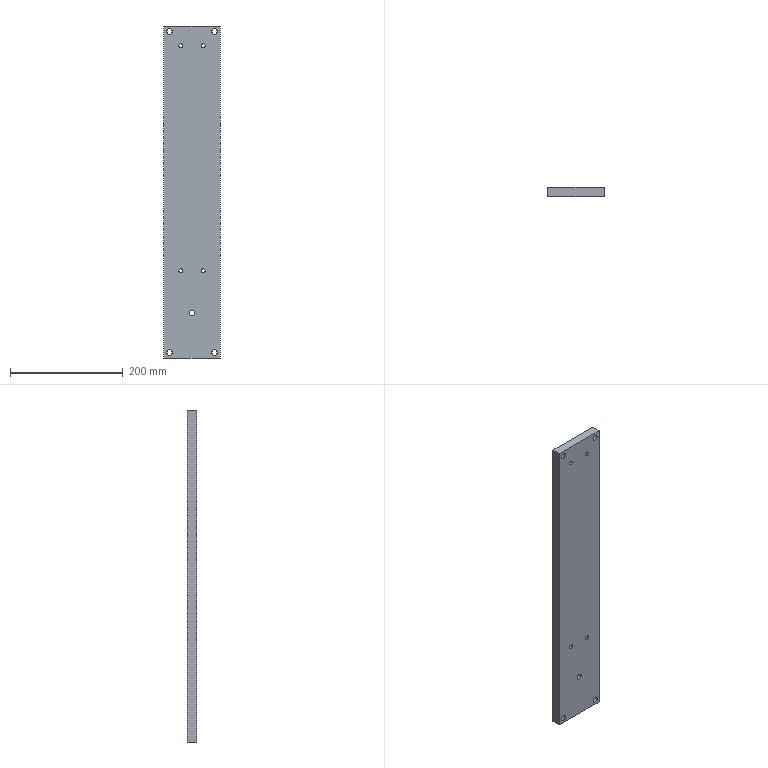Component | SolidWorks | TractionBasePlate-2 | 1 solid | 24 faces | box 100 x 16 x 590 mm | volume 935254 mm3 | cylinder 18 | plane 6 | commonest cylinder face diameters 10 x10 7 x8
build123d program:
from build123d import *

# Parameters (mm, degrees)
SKETCH1_W              = 590
SKETCH1_H              = 100
SKETCH1_R              = 5
SKETCH1_R_2            = 3.5
EXTRUDE1_DEPTH         = 16
M10_TAPPED_HOLE1_D     = 10
M10_TAPPED_HOLE1_DEPTH = 27.5
M10_TAPPED_HOLE1_TIP   = 3.004


with BuildPart() as part:
    # Sketch1 → Extrude1 (new body)
    with BuildSketch(Plane(origin=(0, 0, 0), x_dir=(1, 0, 0), z_dir=(0, 1, 0))):
        Rectangle(SKETCH1_W, SKETCH1_H)
        with Locations(Location((-285, 40, 0), (0, 0, 270))):
            Circle(SKETCH1_R, mode=Mode.SUBTRACT)
        with Locations(Location((-285, -40, 0), (0, 0, 270))):
            Circle(SKETCH1_R, mode=Mode.SUBTRACT)
        with Locations(Location((285, 40, 0), (0, 0, 270))):
            Circle(SKETCH1_R, mode=Mode.SUBTRACT)
        with Locations(Location((285, -40, 0), (0, 0, 270))):
            Circle(SKETCH1_R, mode=Mode.SUBTRACT)
        with Locations(Location((-260, 20, 0), (0, 0, 270))):
            Circle(SKETCH1_R_2, mode=Mode.SUBTRACT)
        with Locations(Location((-260, -20, 0), (0, 0, 270))):
            Circle(SKETCH1_R_2, mode=Mode.SUBTRACT)
        with Locations(Location((140, 20, 0), (0, 0, 270))):
            Circle(SKETCH1_R_2, mode=Mode.SUBTRACT)
        with Locations(Location((140, -20, 0), (0, 0, 270))):
            Circle(SKETCH1_R_2, mode=Mode.SUBTRACT)
    extrude(amount=EXTRUDE1_DEPTH)

    # M10 Tapped Hole1
    with Locations(Plane(origin=(0, 16, 0), x_dir=(-1, 0, 0), z_dir=(0, 1, 0))):
        with Locations((-215, 0)):
            Hole(M10_TAPPED_HOLE1_D / 2, depth=M10_TAPPED_HOLE1_DEPTH)
            with Locations((0, 0, -(M10_TAPPED_HOLE1_DEPTH + M10_TAPPED_HOLE1_TIP / 2))):  # 118° drill point
                Cone(0, M10_TAPPED_HOLE1_D / 2, M10_TAPPED_HOLE1_TIP, mode=Mode.SUBTRACT)


solid = part.part

# Placed as in the assembly
solid = solid.moved(Location((250.216, 370.983, 6.5), (0, 90, 0)))
STEP:
#1=CARTESIAN_POINT('',(9.654,14.606,-8.209));
#2=VERTEX_POINT('',#1);
#3=CARTESIAN_POINT('',(10.048,14.606,-8.209));
#4=VERTEX_POINT('',#3);
#5=CARTESIAN_POINT('',(9.851,14.606,-8.209));
#6=DIRECTION('',(0.,1.,0.));
#7=DIRECTION('',(1.,0.,0.));
#8=AXIS2_PLACEMENT_3D('',#5,#6,#7);
#9=CIRCLE('',#8,0.1969);
#10=EDGE_CURVE('',#2,#4,#9,.T.);
#11=ORIENTED_EDGE('',*,*,#10,.F.);
#12=CARTESIAN_POINT('',(9.654,15.236,-8.209));
#13=VERTEX_POINT('',#12);
#14=CARTESIAN_POINT('',(9.654,15.236,-8.209));
#15=DIRECTION('',(0.,1.,0.));
#16=VECTOR('',#15,39.37);
#17=LINE('',#14,#16);
#18=EDGE_CURVE('',#2,#13,#17,.T.);
#19=ORIENTED_EDGE('',*,*,#18,.T.);
#20=CARTESIAN_POINT('',(10.048,15.236,-8.209));
#21=VERTEX_POINT('',#20);
#22=CARTESIAN_POINT('',(9.851,15.236,-8.209));
#23=DIRECTION('',(0.,1.,0.));
#24=DIRECTION('',(1.,0.,0.));
#25=AXIS2_PLACEMENT_3D('',#22,#23,#24);
#26=CIRCLE('',#25,0.1969);
#27=EDGE_CURVE('',#13,#21,#26,.T.);
#28=ORIENTED_EDGE('',*,*,#27,.T.);
#29=CARTESIAN_POINT('',(10.048,15.236,-8.209));
#30=DIRECTION('',(0.,1.,0.));
#31=VECTOR('',#30,39.37);
#32=LINE('',#29,#31);
#33=EDGE_CURVE('',#4,#21,#32,.T.);
#34=ORIENTED_EDGE('',*,*,#33,.F.);
#35=EDGE_LOOP('',(#11,#19,#28,#34));
#36=FACE_OUTER_BOUND('',#35,.T.);
#37=CARTESIAN_POINT('',(9.851,15.236,-8.209));
#38=DIRECTION('',(0.,1.,0.));
#39=DIRECTION('',(1.,0.,0.));
#40=AXIS2_PLACEMENT_3D('',#37,#38,#39);
#41=CYLINDRICAL_SURFACE('',#40,0.1969);
#42=ADVANCED_FACE('',(#36),#41,.F.);
#43=CARTESIAN_POINT('',(10.501,15.236,-5.256));
#44=VERTEX_POINT('',#43);
#45=CARTESIAN_POINT('',(10.776,15.236,-5.256));
#46=VERTEX_POINT('',#45);
#47=CARTESIAN_POINT('',(10.638,15.236,-5.256));
#48=DIRECTION('',(0.,1.,0.));
#49=DIRECTION('',(1.,0.,0.));
#50=AXIS2_PLACEMENT_3D('',#47,#48,#49);
#51=CIRCLE('',#50,0.1378);
#52=EDGE_CURVE('',#44,#46,#51,.T.);
#53=ORIENTED_EDGE('',*,*,#52,.T.);
#54=CARTESIAN_POINT('',(10.776,14.606,-5.256));
#55=VERTEX_POINT('',#54);
#56=CARTESIAN_POINT('',(10.776,15.236,-5.256));
#57=DIRECTION('',(0.,-1.,0.));
#58=VECTOR('',#57,39.37);
#59=LINE('',#56,#58);
#60=EDGE_CURVE('',#46,#55,#59,.T.);
#61=ORIENTED_EDGE('',*,*,#60,.T.);
#62=CARTESIAN_POINT('',(10.501,14.606,-5.256));
#63=VERTEX_POINT('',#62);
#64=CARTESIAN_POINT('',(10.638,14.606,-5.256));
#65=DIRECTION('',(0.,1.,0.));
#66=DIRECTION('',(1.,0.,0.));
#67=AXIS2_PLACEMENT_3D('',#64,#65,#66);
#68=CIRCLE('',#67,0.1378);
#69=EDGE_CURVE('',#63,#55,#68,.T.);
#70=ORIENTED_EDGE('',*,*,#69,.F.);
#71=CARTESIAN_POINT('',(10.501,15.236,-5.256));
#72=DIRECTION('',(0.,-1.,0.));
#73=VECTOR('',#72,39.37);
#74=LINE('',#71,#73);
#75=EDGE_CURVE('',#44,#63,#74,.T.);
#76=ORIENTED_EDGE('',*,*,#75,.F.);
#77=EDGE_LOOP('',(#53,#61,#70,#76));
#78=FACE_OUTER_BOUND('',#77,.T.);
#79=CARTESIAN_POINT('',(10.638,15.236,-5.256));
#80=DIRECTION('',(0.,-1.,0.));
#81=DIRECTION('',(-1.,0.,0.));
#82=AXIS2_PLACEMENT_3D('',#79,#80,#81);
#83=CYLINDRICAL_SURFACE('',#82,0.1378);
#84=ADVANCED_FACE('',(#78),#83,.F.);
#85=CARTESIAN_POINT('',(8.926,15.236,-5.256));
#86=VERTEX_POINT('',#85);
#87=CARTESIAN_POINT('',(9.201,15.236,-5.256));
#88=VERTEX_POINT('',#87);
#89=CARTESIAN_POINT('',(9.064,15.236,-5.256));
#90=DIRECTION('',(0.,1.,0.));
#91=DIRECTION('',(1.,0.,0.));
#92=AXIS2_PLACEMENT_3D('',#89,#90,#91);
#93=CIRCLE('',#92,0.1378);
#94=EDGE_CURVE('',#86,#88,#93,.T.);
#95=ORIENTED_EDGE('',*,*,#94,.T.);
#96=CARTESIAN_POINT('',(9.201,14.606,-5.256));
#97=VERTEX_POINT('',#96);
#98=CARTESIAN_POINT('',(9.201,15.236,-5.256));
#99=DIRECTION('',(0.,-1.,0.));
#100=VECTOR('',#99,39.37);
#101=LINE('',#98,#100);
#102=EDGE_CURVE('',#88,#97,#101,.T.);
#103=ORIENTED_EDGE('',*,*,#102,.T.);
#104=CARTESIAN_POINT('',(8.926,14.606,-5.256));
#105=VERTEX_POINT('',#104);
#106=CARTESIAN_POINT('',(9.064,14.606,-5.256));
#107=DIRECTION('',(0.,1.,0.));
#108=DIRECTION('',(1.,0.,0.));
#109=AXIS2_PLACEMENT_3D('',#106,#107,#108);
#110=CIRCLE('',#109,0.1378);
#111=EDGE_CURVE('',#105,#97,#110,.T.);
#112=ORIENTED_EDGE('',*,*,#111,.F.);
#113=CARTESIAN_POINT('',(8.926,15.236,-5.256));
#114=DIRECTION('',(0.,-1.,0.));
#115=VECTOR('',#114,39.37);
#116=LINE('',#113,#115);
#117=EDGE_CURVE('',#86,#105,#116,.T.);
#118=ORIENTED_EDGE('',*,*,#117,.F.);
#119=EDGE_LOOP('',(#95,#103,#112,#118));
#120=FACE_OUTER_BOUND('',#119,.T.);
#121=CARTESIAN_POINT('',(9.064,15.236,-5.256));
#122=DIRECTION('',(0.,-1.,0.));
#123=DIRECTION('',(-1.,0.,0.));
#124=AXIS2_PLACEMENT_3D('',#121,#122,#123);
#125=CYLINDRICAL_SURFACE('',#124,0.1378);
#126=ADVANCED_FACE('',(#120),#125,.F.);
#127=CARTESIAN_POINT('',(10.501,15.236,10.492));
#128=VERTEX_POINT('',#127);
#129=CARTESIAN_POINT('',(10.776,15.236,10.492));
#130=VERTEX_POINT('',#129);
#131=CARTESIAN_POINT('',(10.638,15.236,10.492));
#132=DIRECTION('',(0.,1.,0.));
#133=DIRECTION('',(1.,0.,0.));
#134=AXIS2_PLACEMENT_3D('',#131,#132,#133);
#135=CIRCLE('',#134,0.1378);
#136=EDGE_CURVE('',#128,#130,#135,.T.);
#137=ORIENTED_EDGE('',*,*,#136,.T.);
#138=CARTESIAN_POINT('',(10.776,14.606,10.492));
#139=VERTEX_POINT('',#138);
#140=CARTESIAN_POINT('',(10.776,15.236,10.492));
#141=DIRECTION('',(0.,-1.,0.));
#142=VECTOR('',#141,39.37);
#143=LINE('',#140,#142);
#144=EDGE_CURVE('',#130,#139,#143,.T.);
#145=ORIENTED_EDGE('',*,*,#144,.T.);
#146=CARTESIAN_POINT('',(10.501,14.606,10.492));
#147=VERTEX_POINT('',#146);
#148=CARTESIAN_POINT('',(10.638,14.606,10.492));
#149=DIRECTION('',(0.,1.,0.));
#150=DIRECTION('',(1.,0.,0.));
#151=AXIS2_PLACEMENT_3D('',#148,#149,#150);
#152=CIRCLE('',#151,0.1378);
#153=EDGE_CURVE('',#147,#139,#152,.T.);
#154=ORIENTED_EDGE('',*,*,#153,.F.);
#155=CARTESIAN_POINT('',(10.501,15.236,10.492));
#156=DIRECTION('',(0.,-1.,0.));
#157=VECTOR('',#156,39.37);
#158=LINE('',#155,#157);
#159=EDGE_CURVE('',#128,#147,#158,.T.);
#160=ORIENTED_EDGE('',*,*,#159,.F.);
#161=EDGE_LOOP('',(#137,#145,#154,#160));
#162=FACE_OUTER_BOUND('',#161,.T.);
#163=CARTESIAN_POINT('',(10.638,15.236,10.492));
#164=DIRECTION('',(0.,-1.,0.));
#165=DIRECTION('',(-1.,0.,0.));
#166=AXIS2_PLACEMENT_3D('',#163,#164,#165);
#167=CYLINDRICAL_SURFACE('',#166,0.1378);
#168=ADVANCED_FACE('',(#162),#167,.F.);
#169=CARTESIAN_POINT('',(8.926,15.236,10.492));
#170=VERTEX_POINT('',#169);
#171=CARTESIAN_POINT('',(9.201,15.236,10.492));
#172=VERTEX_POINT('',#171);
#173=CARTESIAN_POINT('',(9.064,15.236,10.492));
#174=DIRECTION('',(0.,1.,0.));
#175=DIRECTION('',(1.,0.,0.));
#176=AXIS2_PLACEMENT_3D('',#173,#174,#175);
#177=CIRCLE('',#176,0.1378);
#178=EDGE_CURVE('',#170,#172,#177,.T.);
#179=ORIENTED_EDGE('',*,*,#178,.T.);
#180=CARTESIAN_POINT('',(9.201,14.606,10.492));
#181=VERTEX_POINT('',#180);
#182=CARTESIAN_POINT('',(9.201,15.236,10.492));
#183=DIRECTION('',(0.,-1.,0.));
#184=VECTOR('',#183,39.37);
#185=LINE('',#182,#184);
#186=EDGE_CURVE('',#172,#181,#185,.T.);
#187=ORIENTED_EDGE('',*,*,#186,.T.);
#188=CARTESIAN_POINT('',(8.926,14.606,10.492));
#189=VERTEX_POINT('',#188);
#190=CARTESIAN_POINT('',(9.064,14.606,10.492));
#191=DIRECTION('',(0.,1.,0.));
#192=DIRECTION('',(1.,0.,0.));
#193=AXIS2_PLACEMENT_3D('',#190,#191,#192);
#194=CIRCLE('',#193,0.1378);
#195=EDGE_CURVE('',#189,#181,#194,.T.);
#196=ORIENTED_EDGE('',*,*,#195,.F.);
#197=CARTESIAN_POINT('',(8.926,15.236,10.492));
#198=DIRECTION('',(0.,-1.,0.));
#199=VECTOR('',#198,39.37);
#200=LINE('',#197,#199);
#201=EDGE_CURVE('',#170,#189,#200,.T.);
#202=ORIENTED_EDGE('',*,*,#201,.F.);
#203=EDGE_LOOP('',(#179,#187,#196,#202));
#204=FACE_OUTER_BOUND('',#203,.T.);
#205=CARTESIAN_POINT('',(9.064,15.236,10.492));
#206=DIRECTION('',(0.,-1.,0.));
#207=DIRECTION('',(-1.,0.,0.));
#208=AXIS2_PLACEMENT_3D('',#205,#206,#207);
#209=CYLINDRICAL_SURFACE('',#208,0.1378);
#210=ADVANCED_FACE('',(#204),#209,.F.);
#211=CARTESIAN_POINT('',(11.229,15.236,-10.965));
#212=VERTEX_POINT('',#211);
#213=CARTESIAN_POINT('',(11.623,15.236,-10.965));
#214=VERTEX_POINT('',#213);
#215=CARTESIAN_POINT('',(11.426,15.236,-10.965));
#216=DIRECTION('',(0.,1.,0.));
#217=DIRECTION('',(1.,0.,0.));
#218=AXIS2_PLACEMENT_3D('',#215,#216,#217);
#219=CIRCLE('',#218,0.1969);
#220=EDGE_CURVE('',#212,#214,#219,.T.);
#221=ORIENTED_EDGE('',*,*,#220,.T.);
#222=CARTESIAN_POINT('',(11.623,14.606,-10.965));
#223=VERTEX_POINT('',#222);
#224=CARTESIAN_POINT('',(11.623,15.236,-10.965));
#225=DIRECTION('',(0.,-1.,0.));
#226=VECTOR('',#225,39.37);
#227=LINE('',#224,#226);
#228=EDGE_CURVE('',#214,#223,#227,.T.);
#229=ORIENTED_EDGE('',*,*,#228,.T.);
#230=CARTESIAN_POINT('',(11.229,14.606,-10.965));
#231=VERTEX_POINT('',#230);
#232=CARTESIAN_POINT('',(11.426,14.606,-10.965));
#233=DIRECTION('',(0.,1.,0.));
#234=DIRECTION('',(1.,0.,0.));
#235=AXIS2_PLACEMENT_3D('',#232,#233,#234);
#236=CIRCLE('',#235,0.1969);
#237=EDGE_CURVE('',#231,#223,#236,.T.);
#238=ORIENTED_EDGE('',*,*,#237,.F.);
#239=CARTESIAN_POINT('',(11.229,15.236,-10.965));
#240=DIRECTION('',(0.,-1.,0.));
#241=VECTOR('',#240,39.37);
#242=LINE('',#239,#241);
#243=EDGE_CURVE('',#212,#231,#242,.T.);
#244=ORIENTED_EDGE('',*,*,#243,.F.);
#245=EDGE_LOOP('',(#221,#229,#238,#244));
#246=FACE_OUTER_BOUND('',#245,.T.);
#247=CARTESIAN_POINT('',(11.426,15.236,-10.965));
#248=DIRECTION('',(0.,-1.,0.));
#249=DIRECTION('',(-1.,0.,0.));
#250=AXIS2_PLACEMENT_3D('',#247,#248,#249);
#251=CYLINDRICAL_SURFACE('',#250,0.1969);
#252=ADVANCED_FACE('',(#246),#251,.F.);
#253=CARTESIAN_POINT('',(8.079,15.236,-10.965));
#254=VERTEX_POINT('',#253);
#255=CARTESIAN_POINT('',(8.473,15.236,-10.965));
#256=VERTEX_POINT('',#255);
#257=CARTESIAN_POINT('',(8.276,15.236,-10.965));
#258=DIRECTION('',(0.,1.,0.));
#259=DIRECTION('',(1.,0.,0.));
#260=AXIS2_PLACEMENT_3D('',#257,#258,#259);
#261=CIRCLE('',#260,0.1969);
#262=EDGE_CURVE('',#254,#256,#261,.T.);
#263=ORIENTED_EDGE('',*,*,#262,.T.);
#264=CARTESIAN_POINT('',(8.473,14.606,-10.965));
#265=VERTEX_POINT('',#264);
#266=CARTESIAN_POINT('',(8.473,15.236,-10.965));
#267=DIRECTION('',(0.,-1.,0.));
#268=VECTOR('',#267,39.37);
#269=LINE('',#266,#268);
#270=EDGE_CURVE('',#256,#265,#269,.T.);
#271=ORIENTED_EDGE('',*,*,#270,.T.);
#272=CARTESIAN_POINT('',(8.079,14.606,-10.965));
#273=VERTEX_POINT('',#272);
#274=CARTESIAN_POINT('',(8.276,14.606,-10.965));
#275=DIRECTION('',(0.,1.,0.));
#276=DIRECTION('',(1.,0.,0.));
#277=AXIS2_PLACEMENT_3D('',#274,#275,#276);
#278=CIRCLE('',#277,0.1969);
#279=EDGE_CURVE('',#273,#265,#278,.T.);
#280=ORIENTED_EDGE('',*,*,#279,.F.);
#281=CARTESIAN_POINT('',(8.079,15.236,-10.965));
#282=DIRECTION('',(0.,-1.,0.));
#283=VECTOR('',#282,39.37);
#284=LINE('',#281,#283);
#285=EDGE_CURVE('',#254,#273,#284,.T.);
#286=ORIENTED_EDGE('',*,*,#285,.F.);
#287=EDGE_LOOP('',(#263,#271,#280,#286));
#288=FACE_OUTER_BOUND('',#287,.T.);
#289=CARTESIAN_POINT('',(8.276,15.236,-10.965));
#290=DIRECTION('',(0.,-1.,0.));
#291=DIRECTION('',(-1.,0.,0.));
#292=AXIS2_PLACEMENT_3D('',#289,#290,#291);
#293=CYLINDRICAL_SURFACE('',#292,0.1969);
#294=ADVANCED_FACE('',(#288),#293,.F.);
#295=CARTESIAN_POINT('',(11.229,15.236,11.476));
#296=VERTEX_POINT('',#295);
#297=CARTESIAN_POINT('',(11.623,15.236,11.476));
#298=VERTEX_POINT('',#297);
#299=CARTESIAN_POINT('',(11.426,15.236,11.476));
#300=DIRECTION('',(0.,1.,0.));
#301=DIRECTION('',(1.,0.,0.));
#302=AXIS2_PLACEMENT_3D('',#299,#300,#301);
#303=CIRCLE('',#302,0.1969);
#304=EDGE_CURVE('',#296,#298,#303,.T.);
#305=ORIENTED_EDGE('',*,*,#304,.T.);
#306=CARTESIAN_POINT('',(11.623,14.606,11.476));
#307=VERTEX_POINT('',#306);
#308=CARTESIAN_POINT('',(11.623,15.236,11.476));
#309=DIRECTION('',(0.,-1.,0.));
#310=VECTOR('',#309,39.37);
#311=LINE('',#308,#310);
#312=EDGE_CURVE('',#298,#307,#311,.T.);
#313=ORIENTED_EDGE('',*,*,#312,.T.);
#314=CARTESIAN_POINT('',(11.229,14.606,11.476));
#315=VERTEX_POINT('',#314);
#316=CARTESIAN_POINT('',(11.426,14.606,11.476));
#317=DIRECTION('',(0.,1.,0.));
#318=DIRECTION('',(1.,0.,0.));
#319=AXIS2_PLACEMENT_3D('',#316,#317,#318);
#320=CIRCLE('',#319,0.1969);
#321=EDGE_CURVE('',#315,#307,#320,.T.);
#322=ORIENTED_EDGE('',*,*,#321,.F.);
#323=CARTESIAN_POINT('',(11.229,15.236,11.476));
#324=DIRECTION('',(0.,-1.,0.));
#325=VECTOR('',#324,39.37);
#326=LINE('',#323,#325);
#327=EDGE_CURVE('',#296,#315,#326,.T.);
#328=ORIENTED_EDGE('',*,*,#327,.F.);
#329=EDGE_LOOP('',(#305,#313,#322,#328));
#330=FACE_OUTER_BOUND('',#329,.T.);
#331=CARTESIAN_POINT('',(11.426,15.236,11.476));
#332=DIRECTION('',(0.,-1.,0.));
#333=DIRECTION('',(-1.,0.,0.));
#334=AXIS2_PLACEMENT_3D('',#331,#332,#333);
#335=CYLINDRICAL_SURFACE('',#334,0.1969);
#336=ADVANCED_FACE('',(#330),#335,.F.);
#337=CARTESIAN_POINT('',(8.079,15.236,11.476));
#338=VERTEX_POINT('',#337);
#339=CARTESIAN_POINT('',(8.473,15.236,11.476));
#340=VERTEX_POINT('',#339);
#341=CARTESIAN_POINT('',(8.276,15.236,11.476));
#342=DIRECTION('',(0.,1.,0.));
#343=DIRECTION('',(1.,0.,0.));
#344=AXIS2_PLACEMENT_3D('',#341,#342,#343);
#345=CIRCLE('',#344,0.1969);
#346=EDGE_CURVE('',#338,#340,#345,.T.);
#347=ORIENTED_EDGE('',*,*,#346,.T.);
#348=CARTESIAN_POINT('',(8.473,14.606,11.476));
#349=VERTEX_POINT('',#348);
#350=CARTESIAN_POINT('',(8.473,15.236,11.476));
#351=DIRECTION('',(0.,-1.,0.));
#352=VECTOR('',#351,39.37);
#353=LINE('',#350,#352);
#354=EDGE_CURVE('',#340,#349,#353,.T.);
#355=ORIENTED_EDGE('',*,*,#354,.T.);
#356=CARTESIAN_POINT('',(8.079,14.606,11.476));
#357=VERTEX_POINT('',#356);
#358=CARTESIAN_POINT('',(8.276,14.606,11.476));
#359=DIRECTION('',(0.,1.,0.));
#360=DIRECTION('',(1.,0.,0.));
#361=AXIS2_PLACEMENT_3D('',#358,#359,#360);
#362=CIRCLE('',#361,0.1969);
#363=EDGE_CURVE('',#357,#349,#362,.T.);
#364=ORIENTED_EDGE('',*,*,#363,.F.);
#365=CARTESIAN_POINT('',(8.079,15.236,11.476));
#366=DIRECTION('',(0.,-1.,0.));
#367=VECTOR('',#366,39.37);
#368=LINE('',#365,#367);
#369=EDGE_CURVE('',#338,#357,#368,.T.);
#370=ORIENTED_EDGE('',*,*,#369,.F.);
#371=EDGE_LOOP('',(#347,#355,#364,#370));
#372=FACE_OUTER_BOUND('',#371,.T.);
#373=CARTESIAN_POINT('',(8.276,15.236,11.476));
#374=DIRECTION('',(0.,-1.,0.));
#375=DIRECTION('',(-1.,0.,0.));
#376=AXIS2_PLACEMENT_3D('',#373,#374,#375);
#377=CYLINDRICAL_SURFACE('',#376,0.1969);
#378=ADVANCED_FACE('',(#372),#377,.F.);
#379=CARTESIAN_POINT('',(9.851,15.236,-8.209));
#380=DIRECTION('',(0.,1.,0.));
#381=DIRECTION('',(1.,0.,0.));
#382=AXIS2_PLACEMENT_3D('',#379,#380,#381);
#383=CIRCLE('',#382,0.1969);
#384=EDGE_CURVE('',#21,#13,#383,.T.);
#385=ORIENTED_EDGE('',*,*,#384,.F.);
#386=ORIENTED_EDGE('',*,*,#27,.F.);
#387=EDGE_LOOP('',(#385,#386));
#388=FACE_BOUND('',#387,.T.);
#389=ORIENTED_EDGE('',*,*,#94,.F.);
#390=CARTESIAN_POINT('',(9.064,15.236,-5.256));
#391=DIRECTION('',(0.,1.,0.));
#392=DIRECTION('',(1.,0.,0.));
#393=AXIS2_PLACEMENT_3D('',#390,#391,#392);
#394=CIRCLE('',#393,0.1378);
#395=EDGE_CURVE('',#88,#86,#394,.T.);
#396=ORIENTED_EDGE('',*,*,#395,.F.);
#397=EDGE_LOOP('',(#389,#396));
#398=FACE_BOUND('',#397,.T.);
#399=ORIENTED_EDGE('',*,*,#178,.F.);
#400=CARTESIAN_POINT('',(9.064,15.236,10.492));
#401=DIRECTION('',(0.,1.,0.));
#402=DIRECTION('',(1.,0.,0.));
#403=AXIS2_PLACEMENT_3D('',#400,#401,#402);
#404=CIRCLE('',#403,0.1378);
#405=EDGE_CURVE('',#172,#170,#404,.T.);
#406=ORIENTED_EDGE('',*,*,#405,.F.);
#407=EDGE_LOOP('',(#399,#406));
#408=FACE_BOUND('',#407,.T.);
#409=ORIENTED_EDGE('',*,*,#262,.F.);
#410=CARTESIAN_POINT('',(8.276,15.236,-10.965));
#411=DIRECTION('',(0.,1.,0.));
#412=DIRECTION('',(1.,0.,0.));
#413=AXIS2_PLACEMENT_3D('',#410,#411,#412);
#414=CIRCLE('',#413,0.1969);
#415=EDGE_CURVE('',#256,#254,#414,.T.);
#416=ORIENTED_EDGE('',*,*,#415,.F.);
#417=EDGE_LOOP('',(#409,#416));
#418=FACE_BOUND('',#417,.T.);
#419=ORIENTED_EDGE('',*,*,#346,.F.);
#420=CARTESIAN_POINT('',(8.276,15.236,11.476));
#421=DIRECTION('',(0.,1.,0.));
#422=DIRECTION('',(1.,0.,0.));
#423=AXIS2_PLACEMENT_3D('',#420,#421,#422);
#424=CIRCLE('',#423,0.1969);
#425=EDGE_CURVE('',#340,#338,#424,.T.);
#426=ORIENTED_EDGE('',*,*,#425,.F.);
#427=EDGE_LOOP('',(#419,#426));
#428=FACE_BOUND('',#427,.T.);
#429=CARTESIAN_POINT('',(7.883,15.236,11.87));
#430=VERTEX_POINT('',#429);
#431=CARTESIAN_POINT('',(11.82,15.236,11.87));
#432=VERTEX_POINT('',#431);
#433=CARTESIAN_POINT('',(7.883,15.236,11.87));
#434=DIRECTION('',(1.,0.,0.));
#435=VECTOR('',#434,39.37);
#436=LINE('',#433,#435);
#437=EDGE_CURVE('',#430,#432,#436,.T.);
#438=ORIENTED_EDGE('',*,*,#437,.T.);
#439=CARTESIAN_POINT('',(11.82,15.236,-11.358));
#440=VERTEX_POINT('',#439);
#441=CARTESIAN_POINT('',(11.82,15.236,11.87));
#442=DIRECTION('',(0.,0.,-1.));
#443=VECTOR('',#442,39.37);
#444=LINE('',#441,#443);
#445=EDGE_CURVE('',#432,#440,#444,.T.);
#446=ORIENTED_EDGE('',*,*,#445,.T.);
#447=CARTESIAN_POINT('',(7.883,15.236,-11.358));
#448=VERTEX_POINT('',#447);
#449=CARTESIAN_POINT('',(7.883,15.236,-11.358));
#450=DIRECTION('',(-1.,0.,0.));
#451=VECTOR('',#450,39.37);
#452=LINE('',#449,#451);
#453=EDGE_CURVE('',#440,#448,#452,.T.);
#454=ORIENTED_EDGE('',*,*,#453,.T.);
#455=CARTESIAN_POINT('',(7.883,15.236,11.87));
#456=DIRECTION('',(0.,0.,1.));
#457=VECTOR('',#456,39.37);
#458=LINE('',#455,#457);
#459=EDGE_CURVE('',#448,#430,#458,.T.);
#460=ORIENTED_EDGE('',*,*,#459,.T.);
#461=EDGE_LOOP('',(#438,#446,#454,#460));
#462=FACE_OUTER_BOUND('',#461,.T.);
#463=ORIENTED_EDGE('',*,*,#304,.F.);
#464=CARTESIAN_POINT('',(11.426,15.236,11.476));
#465=DIRECTION('',(0.,1.,0.));
#466=DIRECTION('',(1.,0.,0.));
#467=AXIS2_PLACEMENT_3D('',#464,#465,#466);
#468=CIRCLE('',#467,0.1969);
#469=EDGE_CURVE('',#298,#296,#468,.T.);
#470=ORIENTED_EDGE('',*,*,#469,.F.);
#471=EDGE_LOOP('',(#463,#470));
#472=FACE_BOUND('',#471,.T.);
#473=ORIENTED_EDGE('',*,*,#220,.F.);
#474=CARTESIAN_POINT('',(11.426,15.236,-10.965));
#475=DIRECTION('',(0.,1.,0.));
#476=DIRECTION('',(1.,0.,0.));
#477=AXIS2_PLACEMENT_3D('',#474,#475,#476);
#478=CIRCLE('',#477,0.1969);
#479=EDGE_CURVE('',#214,#212,#478,.T.);
#480=ORIENTED_EDGE('',*,*,#479,.F.);
#481=EDGE_LOOP('',(#473,#480));
#482=FACE_BOUND('',#481,.T.);
#483=ORIENTED_EDGE('',*,*,#136,.F.);
#484=CARTESIAN_POINT('',(10.638,15.236,10.492));
#485=DIRECTION('',(0.,1.,0.));
#486=DIRECTION('',(1.,0.,0.));
#487=AXIS2_PLACEMENT_3D('',#484,#485,#486);
#488=CIRCLE('',#487,0.1378);
#489=EDGE_CURVE('',#130,#128,#488,.T.);
#490=ORIENTED_EDGE('',*,*,#489,.F.);
#491=EDGE_LOOP('',(#483,#490));
#492=FACE_BOUND('',#491,.T.);
#493=ORIENTED_EDGE('',*,*,#52,.F.);
#494=CARTESIAN_POINT('',(10.638,15.236,-5.256));
#495=DIRECTION('',(0.,1.,0.));
#496=DIRECTION('',(1.,0.,0.));
#497=AXIS2_PLACEMENT_3D('',#494,#495,#496);
#498=CIRCLE('',#497,0.1378);
#499=EDGE_CURVE('',#46,#44,#498,.T.);
#500=ORIENTED_EDGE('',*,*,#499,.F.);
#501=EDGE_LOOP('',(#493,#500));
#502=FACE_BOUND('',#501,.T.);
#503=CARTESIAN_POINT('',(11.82,15.236,11.87));
#504=DIRECTION('',(0.,1.,0.));
#505=DIRECTION('',(1.,0.,0.));
#506=AXIS2_PLACEMENT_3D('',#503,#504,#505);
#507=PLANE('',#506);
#508=ADVANCED_FACE('',(#388,#398,#408,#418,#428,#462,#472,#482,#492,#502),#507,.T.);
#509=CARTESIAN_POINT('',(9.851,14.606,-8.209));
#510=DIRECTION('',(0.,1.,0.));
#511=DIRECTION('',(1.,0.,0.));
#512=AXIS2_PLACEMENT_3D('',#509,#510,#511);
#513=CIRCLE('',#512,0.1969);
#514=EDGE_CURVE('',#4,#2,#513,.T.);
#515=ORIENTED_EDGE('',*,*,#514,.T.);
#516=ORIENTED_EDGE('',*,*,#10,.T.);
#517=EDGE_LOOP('',(#515,#516));
#518=FACE_BOUND('',#517,.T.);
#519=CARTESIAN_POINT('',(7.883,14.606,11.87));
#520=VERTEX_POINT('',#519);
#521=CARTESIAN_POINT('',(11.82,14.606,11.87));
#522=VERTEX_POINT('',#521);
#523=CARTESIAN_POINT('',(7.883,14.606,11.87));
#524=DIRECTION('',(1.,0.,0.));
#525=VECTOR('',#524,39.37);
#526=LINE('',#523,#525);
#527=EDGE_CURVE('',#520,#522,#526,.T.);
#528=ORIENTED_EDGE('',*,*,#527,.F.);
#529=CARTESIAN_POINT('',(7.883,14.606,-11.358));
#530=VERTEX_POINT('',#529);
#531=CARTESIAN_POINT('',(7.883,14.606,11.87));
#532=DIRECTION('',(0.,0.,1.));
#533=VECTOR('',#532,39.37);
#534=LINE('',#531,#533);
#535=EDGE_CURVE('',#530,#520,#534,.T.);
#536=ORIENTED_EDGE('',*,*,#535,.F.);
#537=CARTESIAN_POINT('',(11.82,14.606,-11.358));
#538=VERTEX_POINT('',#537);
#539=CARTESIAN_POINT('',(7.883,14.606,-11.358));
#540=DIRECTION('',(-1.,0.,0.));
#541=VECTOR('',#540,39.37);
#542=LINE('',#539,#541);
#543=EDGE_CURVE('',#538,#530,#542,.T.);
#544=ORIENTED_EDGE('',*,*,#543,.F.);
#545=CARTESIAN_POINT('',(11.82,14.606,11.87));
#546=DIRECTION('',(0.,0.,-1.));
#547=VECTOR('',#546,39.37);
#548=LINE('',#545,#547);
#549=EDGE_CURVE('',#522,#538,#548,.T.);
#550=ORIENTED_EDGE('',*,*,#549,.F.);
#551=EDGE_LOOP('',(#528,#536,#544,#550));
#552=FACE_OUTER_BOUND('',#551,.T.);
#553=ORIENTED_EDGE('',*,*,#363,.T.);
#554=CARTESIAN_POINT('',(8.276,14.606,11.476));
#555=DIRECTION('',(0.,1.,0.));
#556=DIRECTION('',(1.,0.,0.));
#557=AXIS2_PLACEMENT_3D('',#554,#555,#556);
#558=CIRCLE('',#557,0.1969);
#559=EDGE_CURVE('',#349,#357,#558,.T.);
#560=ORIENTED_EDGE('',*,*,#559,.T.);
#561=EDGE_LOOP('',(#553,#560));
#562=FACE_BOUND('',#561,.T.);
#563=ORIENTED_EDGE('',*,*,#321,.T.);
#564=CARTESIAN_POINT('',(11.426,14.606,11.476));
#565=DIRECTION('',(0.,1.,0.));
#566=DIRECTION('',(1.,0.,0.));
#567=AXIS2_PLACEMENT_3D('',#564,#565,#566);
#568=CIRCLE('',#567,0.1969);
#569=EDGE_CURVE('',#307,#315,#568,.T.);
#570=ORIENTED_EDGE('',*,*,#569,.T.);
#571=EDGE_LOOP('',(#563,#570));
#572=FACE_BOUND('',#571,.T.);
#573=ORIENTED_EDGE('',*,*,#279,.T.);
#574=CARTESIAN_POINT('',(8.276,14.606,-10.965));
#575=DIRECTION('',(0.,1.,0.));
#576=DIRECTION('',(1.,0.,0.));
#577=AXIS2_PLACEMENT_3D('',#574,#575,#576);
#578=CIRCLE('',#577,0.1969);
#579=EDGE_CURVE('',#265,#273,#578,.T.);
#580=ORIENTED_EDGE('',*,*,#579,.T.);
#581=EDGE_LOOP('',(#573,#580));
#582=FACE_BOUND('',#581,.T.);
#583=ORIENTED_EDGE('',*,*,#237,.T.);
#584=CARTESIAN_POINT('',(11.426,14.606,-10.965));
#585=DIRECTION('',(0.,1.,0.));
#586=DIRECTION('',(1.,0.,0.));
#587=AXIS2_PLACEMENT_3D('',#584,#585,#586);
#588=CIRCLE('',#587,0.1969);
#589=EDGE_CURVE('',#223,#231,#588,.T.);
#590=ORIENTED_EDGE('',*,*,#589,.T.);
#591=EDGE_LOOP('',(#583,#590));
#592=FACE_BOUND('',#591,.T.);
#593=ORIENTED_EDGE('',*,*,#195,.T.);
#594=CARTESIAN_POINT('',(9.064,14.606,10.492));
#595=DIRECTION('',(0.,1.,0.));
#596=DIRECTION('',(1.,0.,0.));
#597=AXIS2_PLACEMENT_3D('',#594,#595,#596);
#598=CIRCLE('',#597,0.1378);
#599=EDGE_CURVE('',#181,#189,#598,.T.);
#600=ORIENTED_EDGE('',*,*,#599,.T.);
#601=EDGE_LOOP('',(#593,#600));
#602=FACE_BOUND('',#601,.T.);
#603=ORIENTED_EDGE('',*,*,#153,.T.);
#604=CARTESIAN_POINT('',(10.638,14.606,10.492));
#605=DIRECTION('',(0.,1.,0.));
#606=DIRECTION('',(1.,0.,0.));
#607=AXIS2_PLACEMENT_3D('',#604,#605,#606);
#608=CIRCLE('',#607,0.1378);
#609=EDGE_CURVE('',#139,#147,#608,.T.);
#610=ORIENTED_EDGE('',*,*,#609,.T.);
#611=EDGE_LOOP('',(#603,#610));
#612=FACE_BOUND('',#611,.T.);
#613=ORIENTED_EDGE('',*,*,#111,.T.);
#614=CARTESIAN_POINT('',(9.064,14.606,-5.256));
#615=DIRECTION('',(0.,1.,0.));
#616=DIRECTION('',(1.,0.,0.));
#617=AXIS2_PLACEMENT_3D('',#614,#615,#616);
#618=CIRCLE('',#617,0.1378);
#619=EDGE_CURVE('',#97,#105,#618,.T.);
#620=ORIENTED_EDGE('',*,*,#619,.T.);
#621=EDGE_LOOP('',(#613,#620));
#622=FACE_BOUND('',#621,.T.);
#623=ORIENTED_EDGE('',*,*,#69,.T.);
#624=CARTESIAN_POINT('',(10.638,14.606,-5.256));
#625=DIRECTION('',(0.,1.,0.));
#626=DIRECTION('',(1.,0.,0.));
#627=AXIS2_PLACEMENT_3D('',#624,#625,#626);
#628=CIRCLE('',#627,0.1378);
#629=EDGE_CURVE('',#55,#63,#628,.T.);
#630=ORIENTED_EDGE('',*,*,#629,.T.);
#631=EDGE_LOOP('',(#623,#630));
#632=FACE_BOUND('',#631,.T.);
#633=CARTESIAN_POINT('',(11.82,14.606,11.87));
#634=DIRECTION('',(0.,1.,0.));
#635=DIRECTION('',(1.,0.,0.));
#636=AXIS2_PLACEMENT_3D('',#633,#634,#635);
#637=PLANE('',#636);
#638=ADVANCED_FACE('',(#518,#552,#562,#572,#582,#592,#602,#612,#622,#632),#637,.F.);
#639=ORIENTED_EDGE('',*,*,#527,.T.);
#640=CARTESIAN_POINT('',(11.82,15.236,11.87));
#641=DIRECTION('',(0.,-1.,0.));
#642=VECTOR('',#641,39.37);
#643=LINE('',#640,#642);
#644=EDGE_CURVE('',#432,#522,#643,.T.);
#645=ORIENTED_EDGE('',*,*,#644,.F.);
#646=ORIENTED_EDGE('',*,*,#437,.F.);
#647=CARTESIAN_POINT('',(7.883,15.236,11.87));
#648=DIRECTION('',(0.,-1.,0.));
#649=VECTOR('',#648,39.37);
#650=LINE('',#647,#649);
#651=EDGE_CURVE('',#430,#520,#650,.T.);
#652=ORIENTED_EDGE('',*,*,#651,.T.);
#653=EDGE_LOOP('',(#639,#645,#646,#652));
#654=FACE_OUTER_BOUND('',#653,.T.);
#655=CARTESIAN_POINT('',(7.883,15.236,11.87));
#656=DIRECTION('',(0.,0.,-1.));
#657=DIRECTION('',(-1.,0.,0.));
#658=AXIS2_PLACEMENT_3D('',#655,#656,#657);
#659=PLANE('',#658);
#660=ADVANCED_FACE('',(#654),#659,.F.);
#661=ORIENTED_EDGE('',*,*,#549,.T.);
#662=CARTESIAN_POINT('',(11.82,15.236,-11.358));
#663=DIRECTION('',(0.,-1.,0.));
#664=VECTOR('',#663,39.37);
#665=LINE('',#662,#664);
#666=EDGE_CURVE('',#440,#538,#665,.T.);
#667=ORIENTED_EDGE('',*,*,#666,.F.);
#668=ORIENTED_EDGE('',*,*,#445,.F.);
#669=ORIENTED_EDGE('',*,*,#644,.T.);
#670=EDGE_LOOP('',(#661,#667,#668,#669));
#671=FACE_OUTER_BOUND('',#670,.T.);
#672=CARTESIAN_POINT('',(11.82,15.236,11.87));
#673=DIRECTION('',(-1.,0.,0.));
#674=DIRECTION('',(0.,0.,1.));
#675=AXIS2_PLACEMENT_3D('',#672,#673,#674);
#676=PLANE('',#675);
#677=ADVANCED_FACE('',(#671),#676,.F.);
#678=ORIENTED_EDGE('',*,*,#543,.T.);
#679=CARTESIAN_POINT('',(7.883,15.236,-11.358));
#680=DIRECTION('',(0.,-1.,0.));
#681=VECTOR('',#680,39.37);
#682=LINE('',#679,#681);
#683=EDGE_CURVE('',#448,#530,#682,.T.);
#684=ORIENTED_EDGE('',*,*,#683,.F.);
#685=ORIENTED_EDGE('',*,*,#453,.F.);
#686=ORIENTED_EDGE('',*,*,#666,.T.);
#687=EDGE_LOOP('',(#678,#684,#685,#686));
#688=FACE_OUTER_BOUND('',#687,.T.);
#689=CARTESIAN_POINT('',(7.883,15.236,-11.358));
#690=DIRECTION('',(0.,0.,1.));
#691=DIRECTION('',(1.,0.,0.));
#692=AXIS2_PLACEMENT_3D('',#689,#690,#691);
#693=PLANE('',#692);
#694=ADVANCED_FACE('',(#688),#693,.F.);
#695=ORIENTED_EDGE('',*,*,#535,.T.);
#696=ORIENTED_EDGE('',*,*,#651,.F.);
#697=ORIENTED_EDGE('',*,*,#459,.F.);
#698=ORIENTED_EDGE('',*,*,#683,.T.);
#699=EDGE_LOOP('',(#695,#696,#697,#698));
#700=FACE_OUTER_BOUND('',#699,.T.);
#701=CARTESIAN_POINT('',(7.883,15.236,11.87));
#702=DIRECTION('',(1.,0.,0.));
#703=DIRECTION('',(0.,0.,-1.));
#704=AXIS2_PLACEMENT_3D('',#701,#702,#703);
#705=PLANE('',#704);
#706=ADVANCED_FACE('',(#700),#705,.F.);
#707=ORIENTED_EDGE('',*,*,#354,.F.);
#708=ORIENTED_EDGE('',*,*,#425,.T.);
#709=ORIENTED_EDGE('',*,*,#369,.T.);
#710=ORIENTED_EDGE('',*,*,#559,.F.);
#711=EDGE_LOOP('',(#707,#708,#709,#710));
#712=FACE_OUTER_BOUND('',#711,.T.);
#713=CARTESIAN_POINT('',(8.276,15.236,11.476));
#714=DIRECTION('',(0.,-1.,0.));
#715=DIRECTION('',(-1.,0.,0.));
#716=AXIS2_PLACEMENT_3D('',#713,#714,#715);
#717=CYLINDRICAL_SURFACE('',#716,0.1969);
#718=ADVANCED_FACE('',(#712),#717,.F.);
#719=ORIENTED_EDGE('',*,*,#312,.F.);
#720=ORIENTED_EDGE('',*,*,#469,.T.);
#721=ORIENTED_EDGE('',*,*,#327,.T.);
#722=ORIENTED_EDGE('',*,*,#569,.F.);
#723=EDGE_LOOP('',(#719,#720,#721,#722));
#724=FACE_OUTER_BOUND('',#723,.T.);
#725=CARTESIAN_POINT('',(11.426,15.236,11.476));
#726=DIRECTION('',(0.,-1.,0.));
#727=DIRECTION('',(-1.,0.,0.));
#728=AXIS2_PLACEMENT_3D('',#725,#726,#727);
#729=CYLINDRICAL_SURFACE('',#728,0.1969);
#730=ADVANCED_FACE('',(#724),#729,.F.);
#731=ORIENTED_EDGE('',*,*,#270,.F.);
#732=ORIENTED_EDGE('',*,*,#415,.T.);
#733=ORIENTED_EDGE('',*,*,#285,.T.);
#734=ORIENTED_EDGE('',*,*,#579,.F.);
#735=EDGE_LOOP('',(#731,#732,#733,#734));
#736=FACE_OUTER_BOUND('',#735,.T.);
#737=CARTESIAN_POINT('',(8.276,15.236,-10.965));
#738=DIRECTION('',(0.,-1.,0.));
#739=DIRECTION('',(-1.,0.,0.));
#740=AXIS2_PLACEMENT_3D('',#737,#738,#739);
#741=CYLINDRICAL_SURFACE('',#740,0.1969);
#742=ADVANCED_FACE('',(#736),#741,.F.);
#743=ORIENTED_EDGE('',*,*,#228,.F.);
#744=ORIENTED_EDGE('',*,*,#479,.T.);
#745=ORIENTED_EDGE('',*,*,#243,.T.);
#746=ORIENTED_EDGE('',*,*,#589,.F.);
#747=EDGE_LOOP('',(#743,#744,#745,#746));
#748=FACE_OUTER_BOUND('',#747,.T.);
#749=CARTESIAN_POINT('',(11.426,15.236,-10.965));
#750=DIRECTION('',(0.,-1.,0.));
#751=DIRECTION('',(-1.,0.,0.));
#752=AXIS2_PLACEMENT_3D('',#749,#750,#751);
#753=CYLINDRICAL_SURFACE('',#752,0.1969);
#754=ADVANCED_FACE('',(#748),#753,.F.);
#755=ORIENTED_EDGE('',*,*,#186,.F.);
#756=ORIENTED_EDGE('',*,*,#405,.T.);
#757=ORIENTED_EDGE('',*,*,#201,.T.);
#758=ORIENTED_EDGE('',*,*,#599,.F.);
#759=EDGE_LOOP('',(#755,#756,#757,#758));
#760=FACE_OUTER_BOUND('',#759,.T.);
#761=CARTESIAN_POINT('',(9.064,15.236,10.492));
#762=DIRECTION('',(0.,-1.,0.));
#763=DIRECTION('',(-1.,0.,0.));
#764=AXIS2_PLACEMENT_3D('',#761,#762,#763);
#765=CYLINDRICAL_SURFACE('',#764,0.1378);
#766=ADVANCED_FACE('',(#760),#765,.F.);
#767=ORIENTED_EDGE('',*,*,#144,.F.);
#768=ORIENTED_EDGE('',*,*,#489,.T.);
#769=ORIENTED_EDGE('',*,*,#159,.T.);
#770=ORIENTED_EDGE('',*,*,#609,.F.);
#771=EDGE_LOOP('',(#767,#768,#769,#770));
#772=FACE_OUTER_BOUND('',#771,.T.);
#773=CARTESIAN_POINT('',(10.638,15.236,10.492));
#774=DIRECTION('',(0.,-1.,0.));
#775=DIRECTION('',(-1.,0.,0.));
#776=AXIS2_PLACEMENT_3D('',#773,#774,#775);
#777=CYLINDRICAL_SURFACE('',#776,0.1378);
#778=ADVANCED_FACE('',(#772),#777,.F.);
#779=ORIENTED_EDGE('',*,*,#102,.F.);
#780=ORIENTED_EDGE('',*,*,#395,.T.);
#781=ORIENTED_EDGE('',*,*,#117,.T.);
#782=ORIENTED_EDGE('',*,*,#619,.F.);
#783=EDGE_LOOP('',(#779,#780,#781,#782));
#784=FACE_OUTER_BOUND('',#783,.T.);
#785=CARTESIAN_POINT('',(9.064,15.236,-5.256));
#786=DIRECTION('',(0.,-1.,0.));
#787=DIRECTION('',(-1.,0.,0.));
#788=AXIS2_PLACEMENT_3D('',#785,#786,#787);
#789=CYLINDRICAL_SURFACE('',#788,0.1378);
#790=ADVANCED_FACE('',(#784),#789,.F.);
#791=ORIENTED_EDGE('',*,*,#60,.F.);
#792=ORIENTED_EDGE('',*,*,#499,.T.);
#793=ORIENTED_EDGE('',*,*,#75,.T.);
#794=ORIENTED_EDGE('',*,*,#629,.F.);
#795=EDGE_LOOP('',(#791,#792,#793,#794));
#796=FACE_OUTER_BOUND('',#795,.T.);
#797=CARTESIAN_POINT('',(10.638,15.236,-5.256));
#798=DIRECTION('',(0.,-1.,0.));
#799=DIRECTION('',(-1.,0.,0.));
#800=AXIS2_PLACEMENT_3D('',#797,#798,#799);
#801=CYLINDRICAL_SURFACE('',#800,0.1378);
#802=ADVANCED_FACE('',(#796),#801,.F.);
#803=ORIENTED_EDGE('',*,*,#18,.F.);
#804=ORIENTED_EDGE('',*,*,#514,.F.);
#805=ORIENTED_EDGE('',*,*,#33,.T.);
#806=ORIENTED_EDGE('',*,*,#384,.T.);
#807=EDGE_LOOP('',(#803,#804,#805,#806));
#808=FACE_OUTER_BOUND('',#807,.T.);
#809=CARTESIAN_POINT('',(9.851,15.236,-8.209));
#810=DIRECTION('',(0.,1.,0.));
#811=DIRECTION('',(1.,0.,0.));
#812=AXIS2_PLACEMENT_3D('',#809,#810,#811);
#813=CYLINDRICAL_SURFACE('',#812,0.1969);
#814=ADVANCED_FACE('',(#808),#813,.F.);
#815=CLOSED_SHELL('',(#42,#84,#126,#168,#210,#252,#294,#336,#378,#508,#638,#660,#677,#694,#706,#718,#730,#742,#754,#766,#778,#790,#802,#814));
#816=MANIFOLD_SOLID_BREP('',#815);
#817=CARTESIAN_POINT('',(0.,0.,0.));
#818=DIRECTION('',(0.,0.,1.));
#819=DIRECTION('',(1.,0.,0.));
#820=AXIS2_PLACEMENT_3D('',#817,#818,#819);
#821=(LENGTH_UNIT()NAMED_UNIT(*)SI_UNIT($,.METRE.));
#822=LENGTH_MEASURE_WITH_UNIT(LENGTH_MEASURE(0.0254),#821);
#823=DIMENSIONAL_EXPONENTS(1.,0.,0.,0.,0.,0.,0.);
#824=(CONVERSION_BASED_UNIT('',#822)LENGTH_UNIT()NAMED_UNIT(#823));
#825=UNCERTAINTY_MEASURE_WITH_UNIT(LENGTH_MEASURE(0.00001),#824,'','');
#826=(NAMED_UNIT(*)PLANE_ANGLE_UNIT()SI_UNIT($,.RADIAN.));
#827=(NAMED_UNIT(*)SI_UNIT($,.STERADIAN.)SOLID_ANGLE_UNIT());
#828=(GEOMETRIC_REPRESENTATION_CONTEXT(3)GLOBAL_UNCERTAINTY_ASSIGNED_CONTEXT((#825))GLOBAL_UNIT_ASSIGNED_CONTEXT((#824,#826,#827))REPRESENTATION_CONTEXT('',''));
#829=ADVANCED_BREP_SHAPE_REPRESENTATION('',(#816,#820),#828);
#830=COLOUR_RGB('',0.7922,0.8196,0.9333);
#831=FILL_AREA_STYLE_COLOUR('',#830);
#832=FILL_AREA_STYLE('',(#831));
#833=SURFACE_STYLE_FILL_AREA(#832);
#834=SURFACE_SIDE_STYLE('',(#833));
#835=SURFACE_STYLE_USAGE(.BOTH.,#834);
#836=PRESENTATION_STYLE_ASSIGNMENT((#835));
#837=STYLED_ITEM('',(#836),#816);
#838=PRESENTATION_LAYER_ASSIGNMENT('','',(#837));
#839=(LENGTH_UNIT()NAMED_UNIT(*)SI_UNIT($,.METRE.));
#840=LENGTH_MEASURE_WITH_UNIT(LENGTH_MEASURE(0.0254),#839);
#841=DIMENSIONAL_EXPONENTS(1.,0.,0.,0.,0.,0.,0.);
#842=(CONVERSION_BASED_UNIT('',#840)LENGTH_UNIT()NAMED_UNIT(#841));
#843=UNCERTAINTY_MEASURE_WITH_UNIT(LENGTH_MEASURE(0.00001),#842,'','');
#844=(NAMED_UNIT(*)PLANE_ANGLE_UNIT()SI_UNIT($,.RADIAN.));
#845=(NAMED_UNIT(*)SI_UNIT($,.STERADIAN.)SOLID_ANGLE_UNIT());
#846=(GEOMETRIC_REPRESENTATION_CONTEXT(3)GLOBAL_UNCERTAINTY_ASSIGNED_CONTEXT((#843))GLOBAL_UNIT_ASSIGNED_CONTEXT((#842,#844,#845))REPRESENTATION_CONTEXT('',''));
#847=MECHANICAL_DESIGN_GEOMETRIC_PRESENTATION_REPRESENTATION('',(#837),#846);